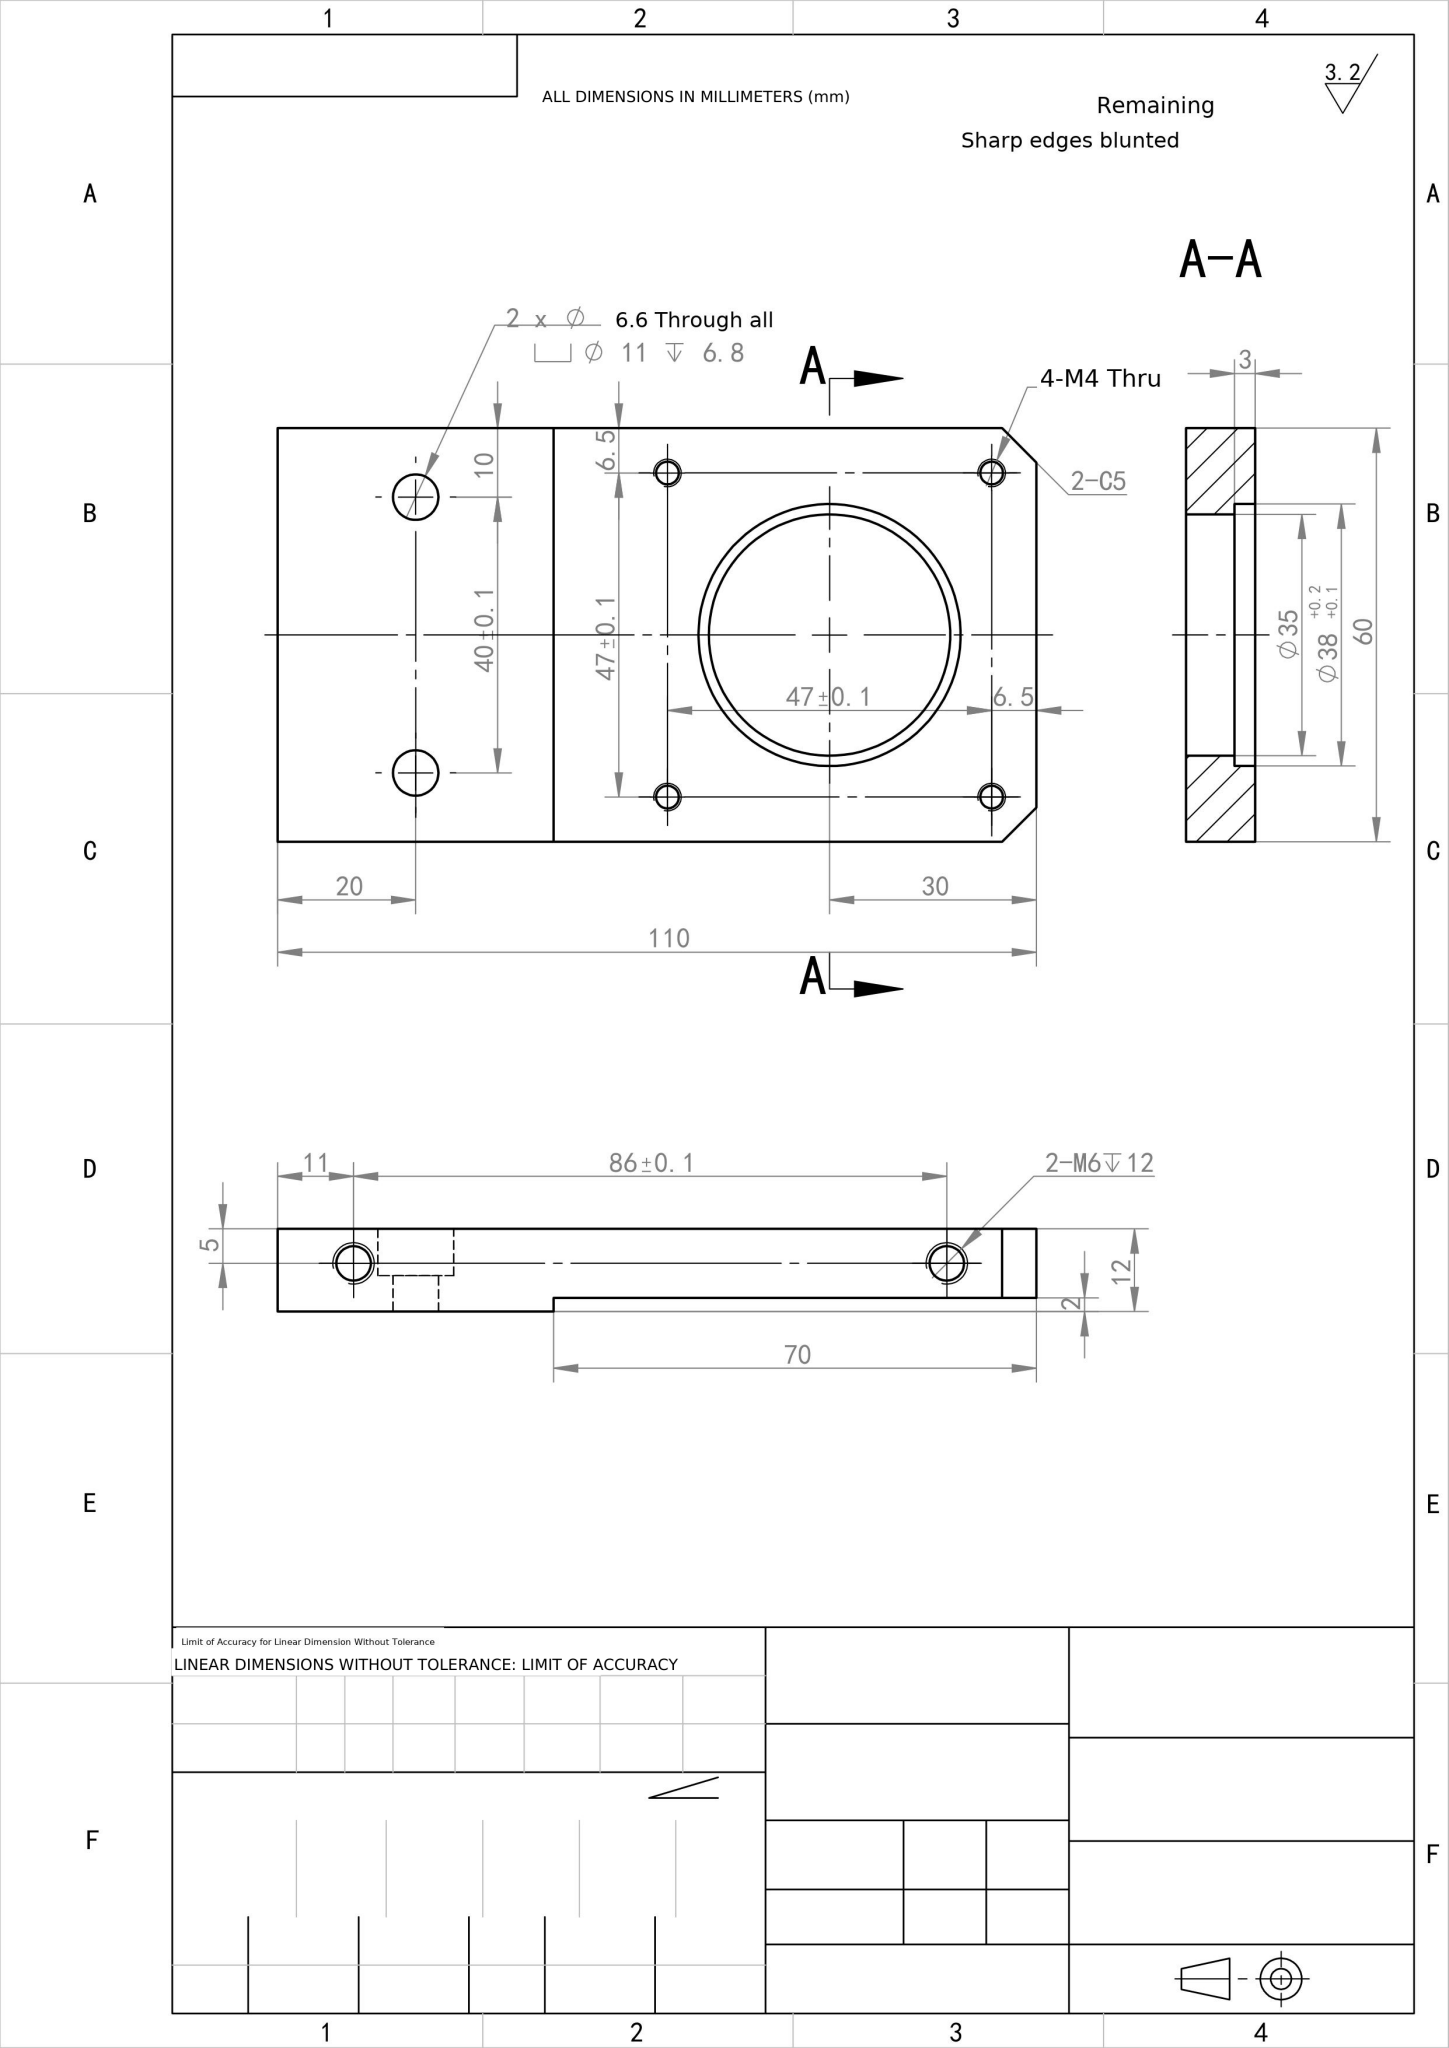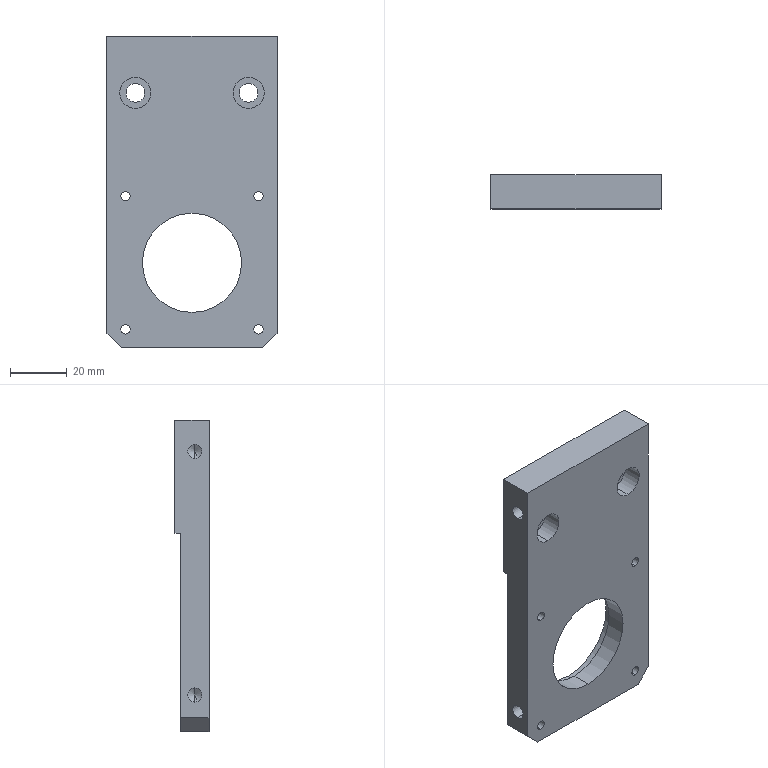Part | NX | mm | 1 solid | 41 faces | box 60 x 12 x 110 mm | volume 57814 mm3 | cylinder 24 | plane 13 | cone 4 | commonest cylinder face diameters 3.3 x8 5 x4 11 x4 6.6 x4 38 x2 35 x2